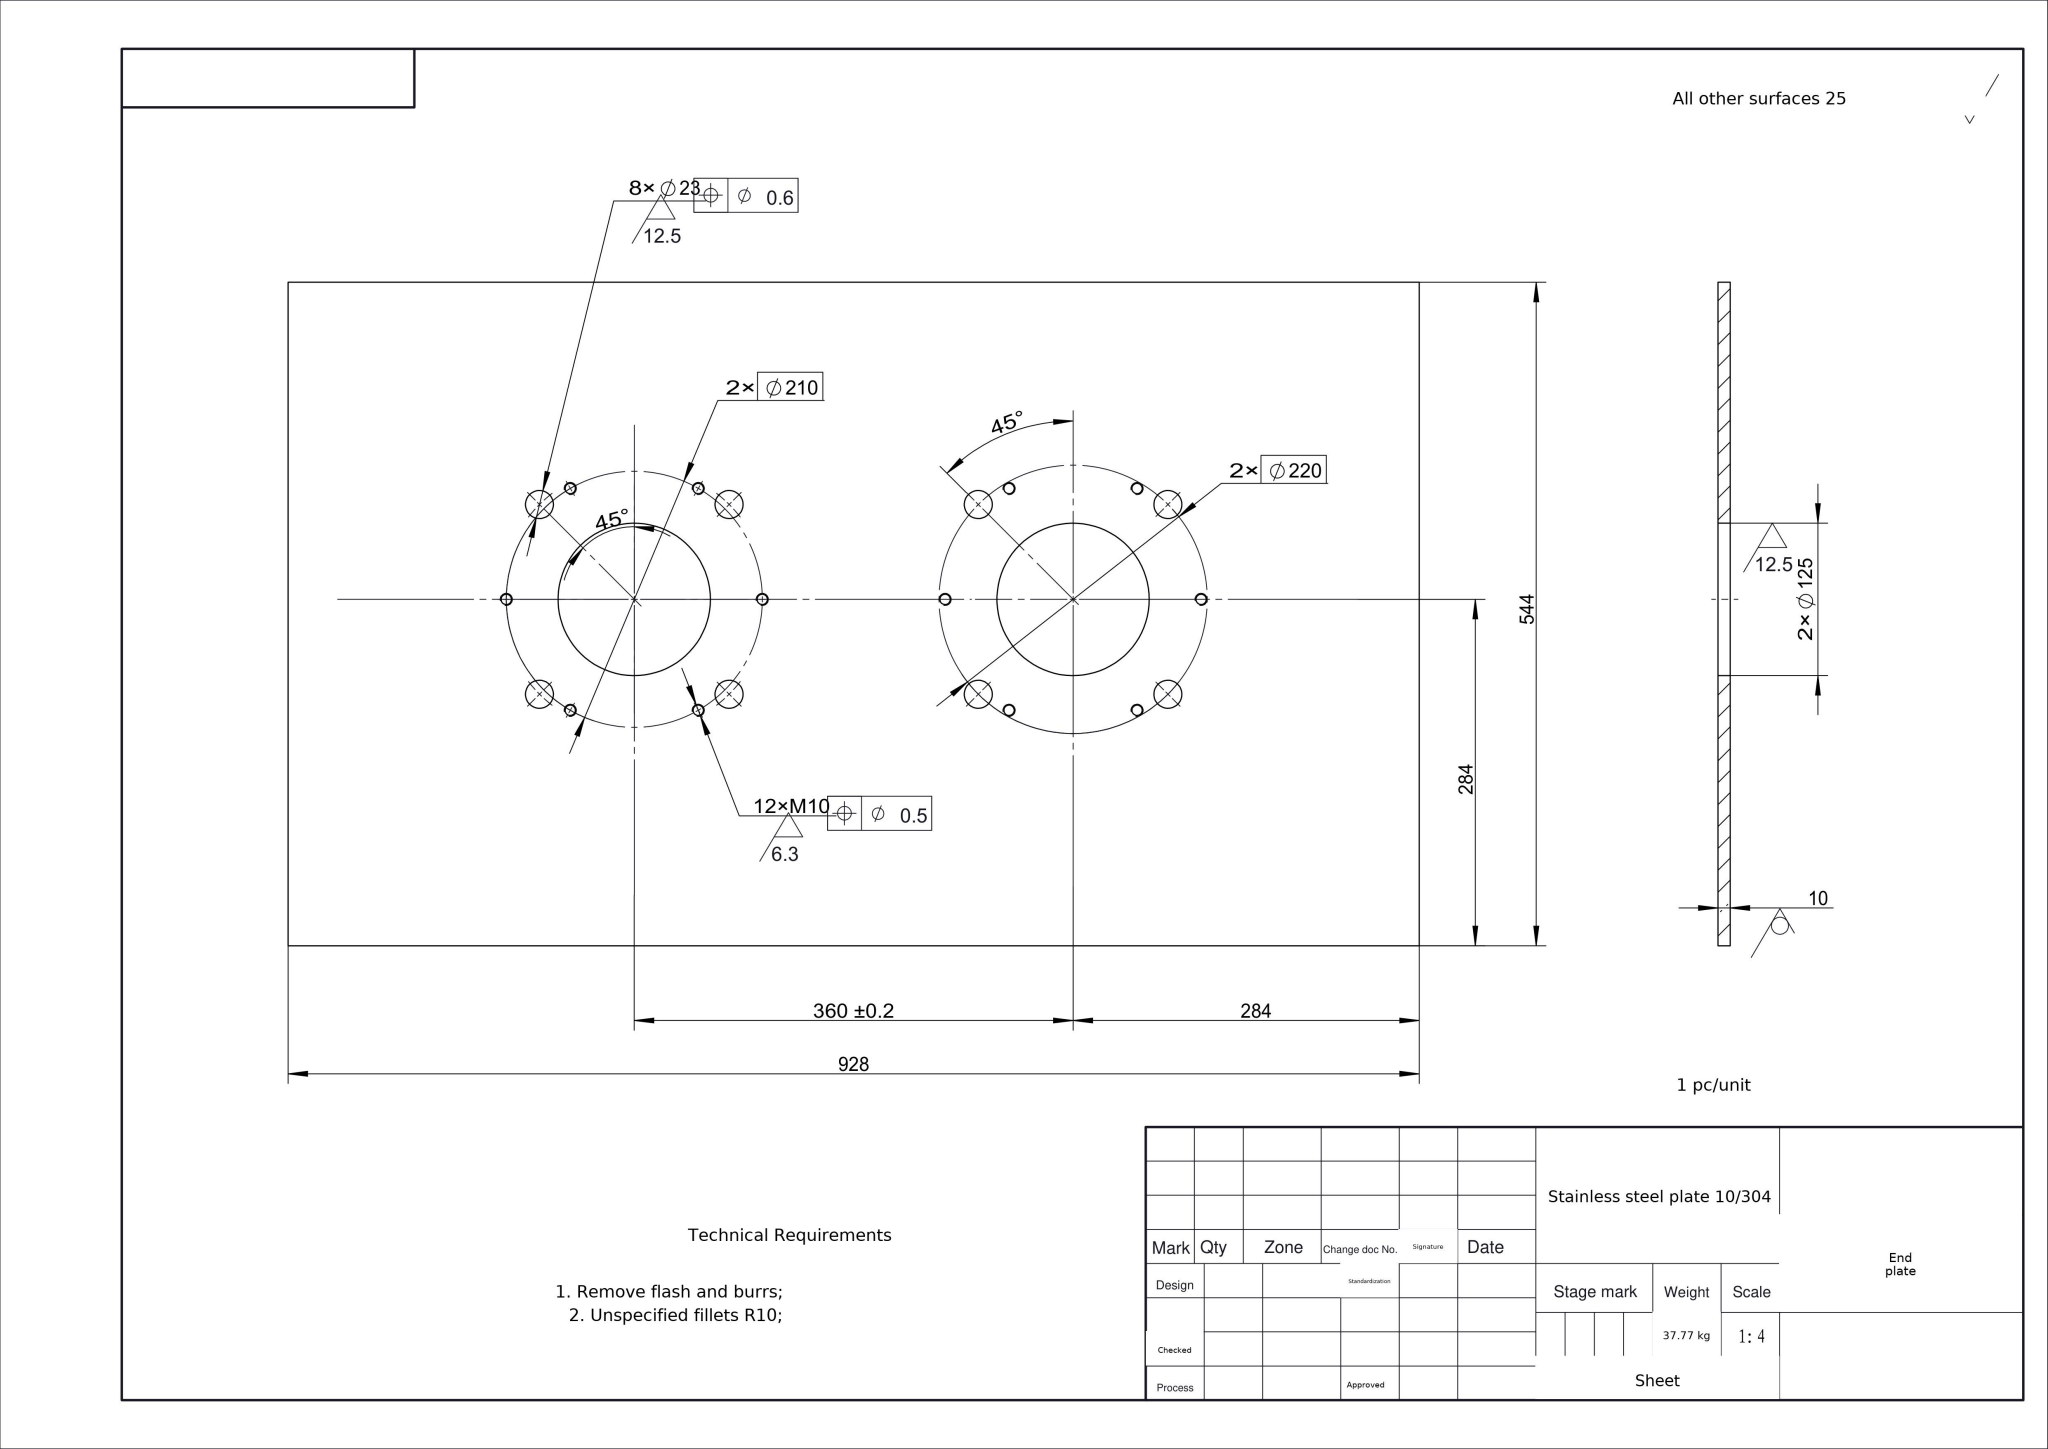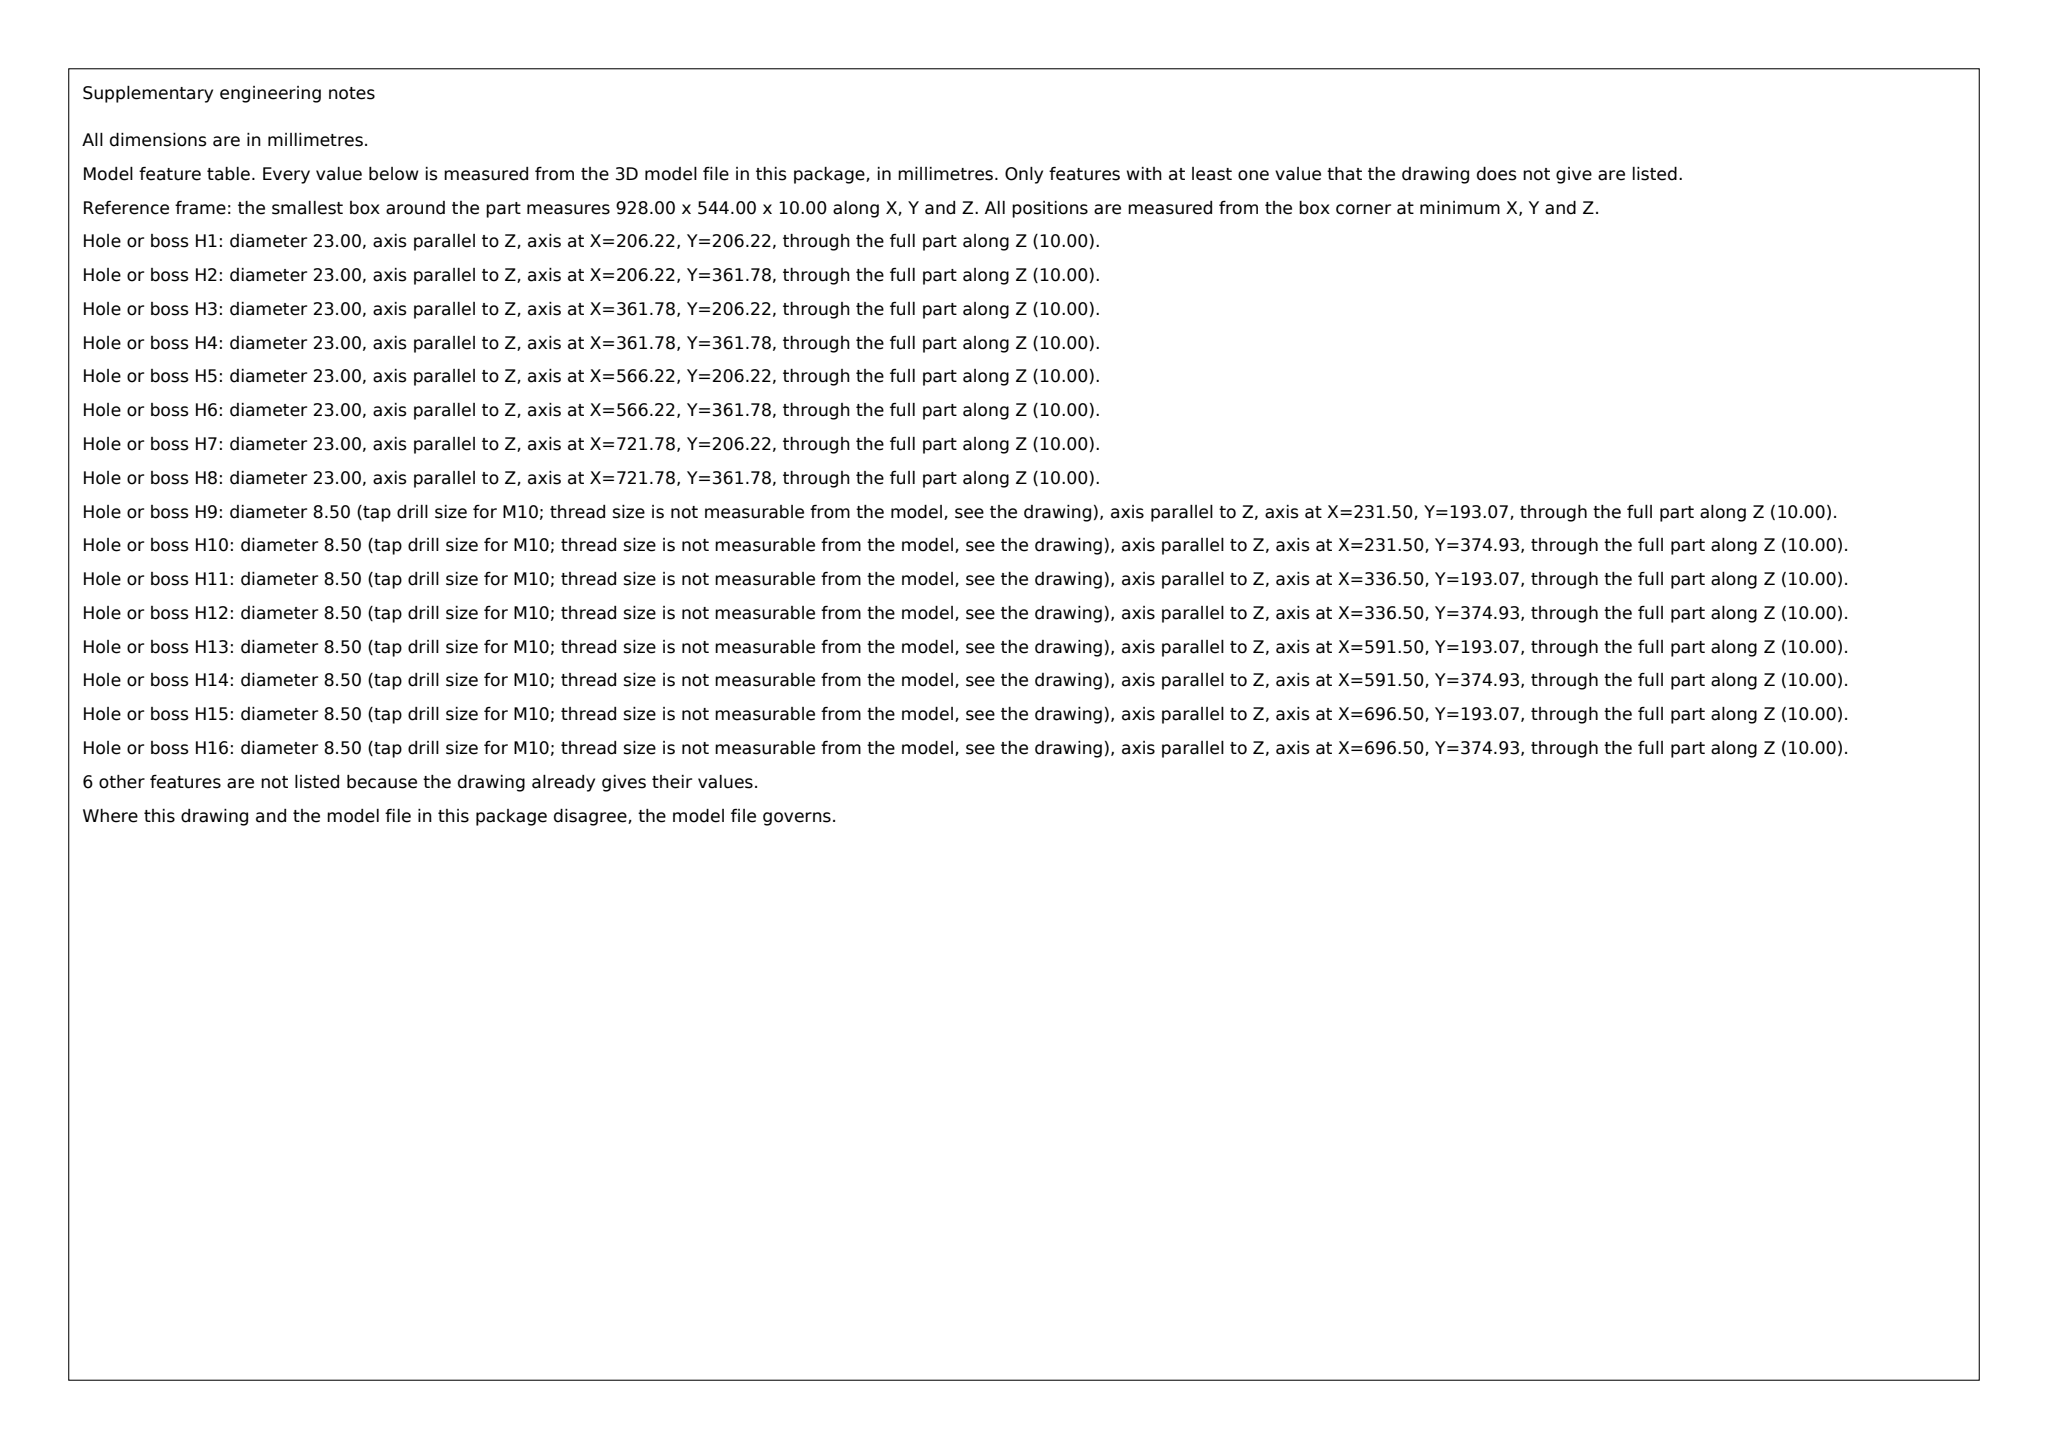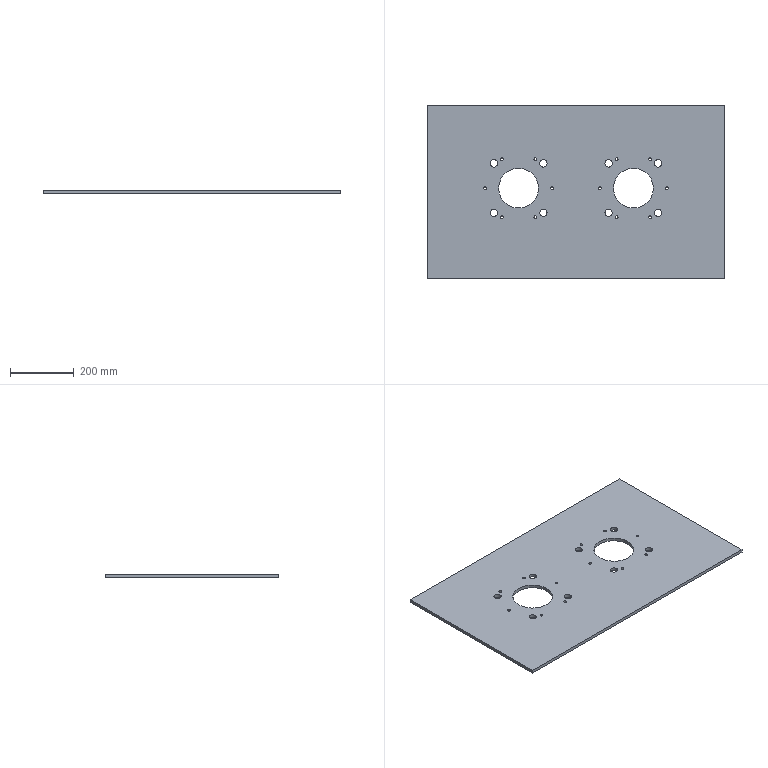Part | SolidWorks | mm | material Stainless steel plate 10/304 | 1 solid | 50 faces | box 928 x 544 x 10 mm | volume 4762836 mm3 | cylinder 44 | plane 6 | commonest cylinder face diameters 8.5 x24 23 x16 125 x4